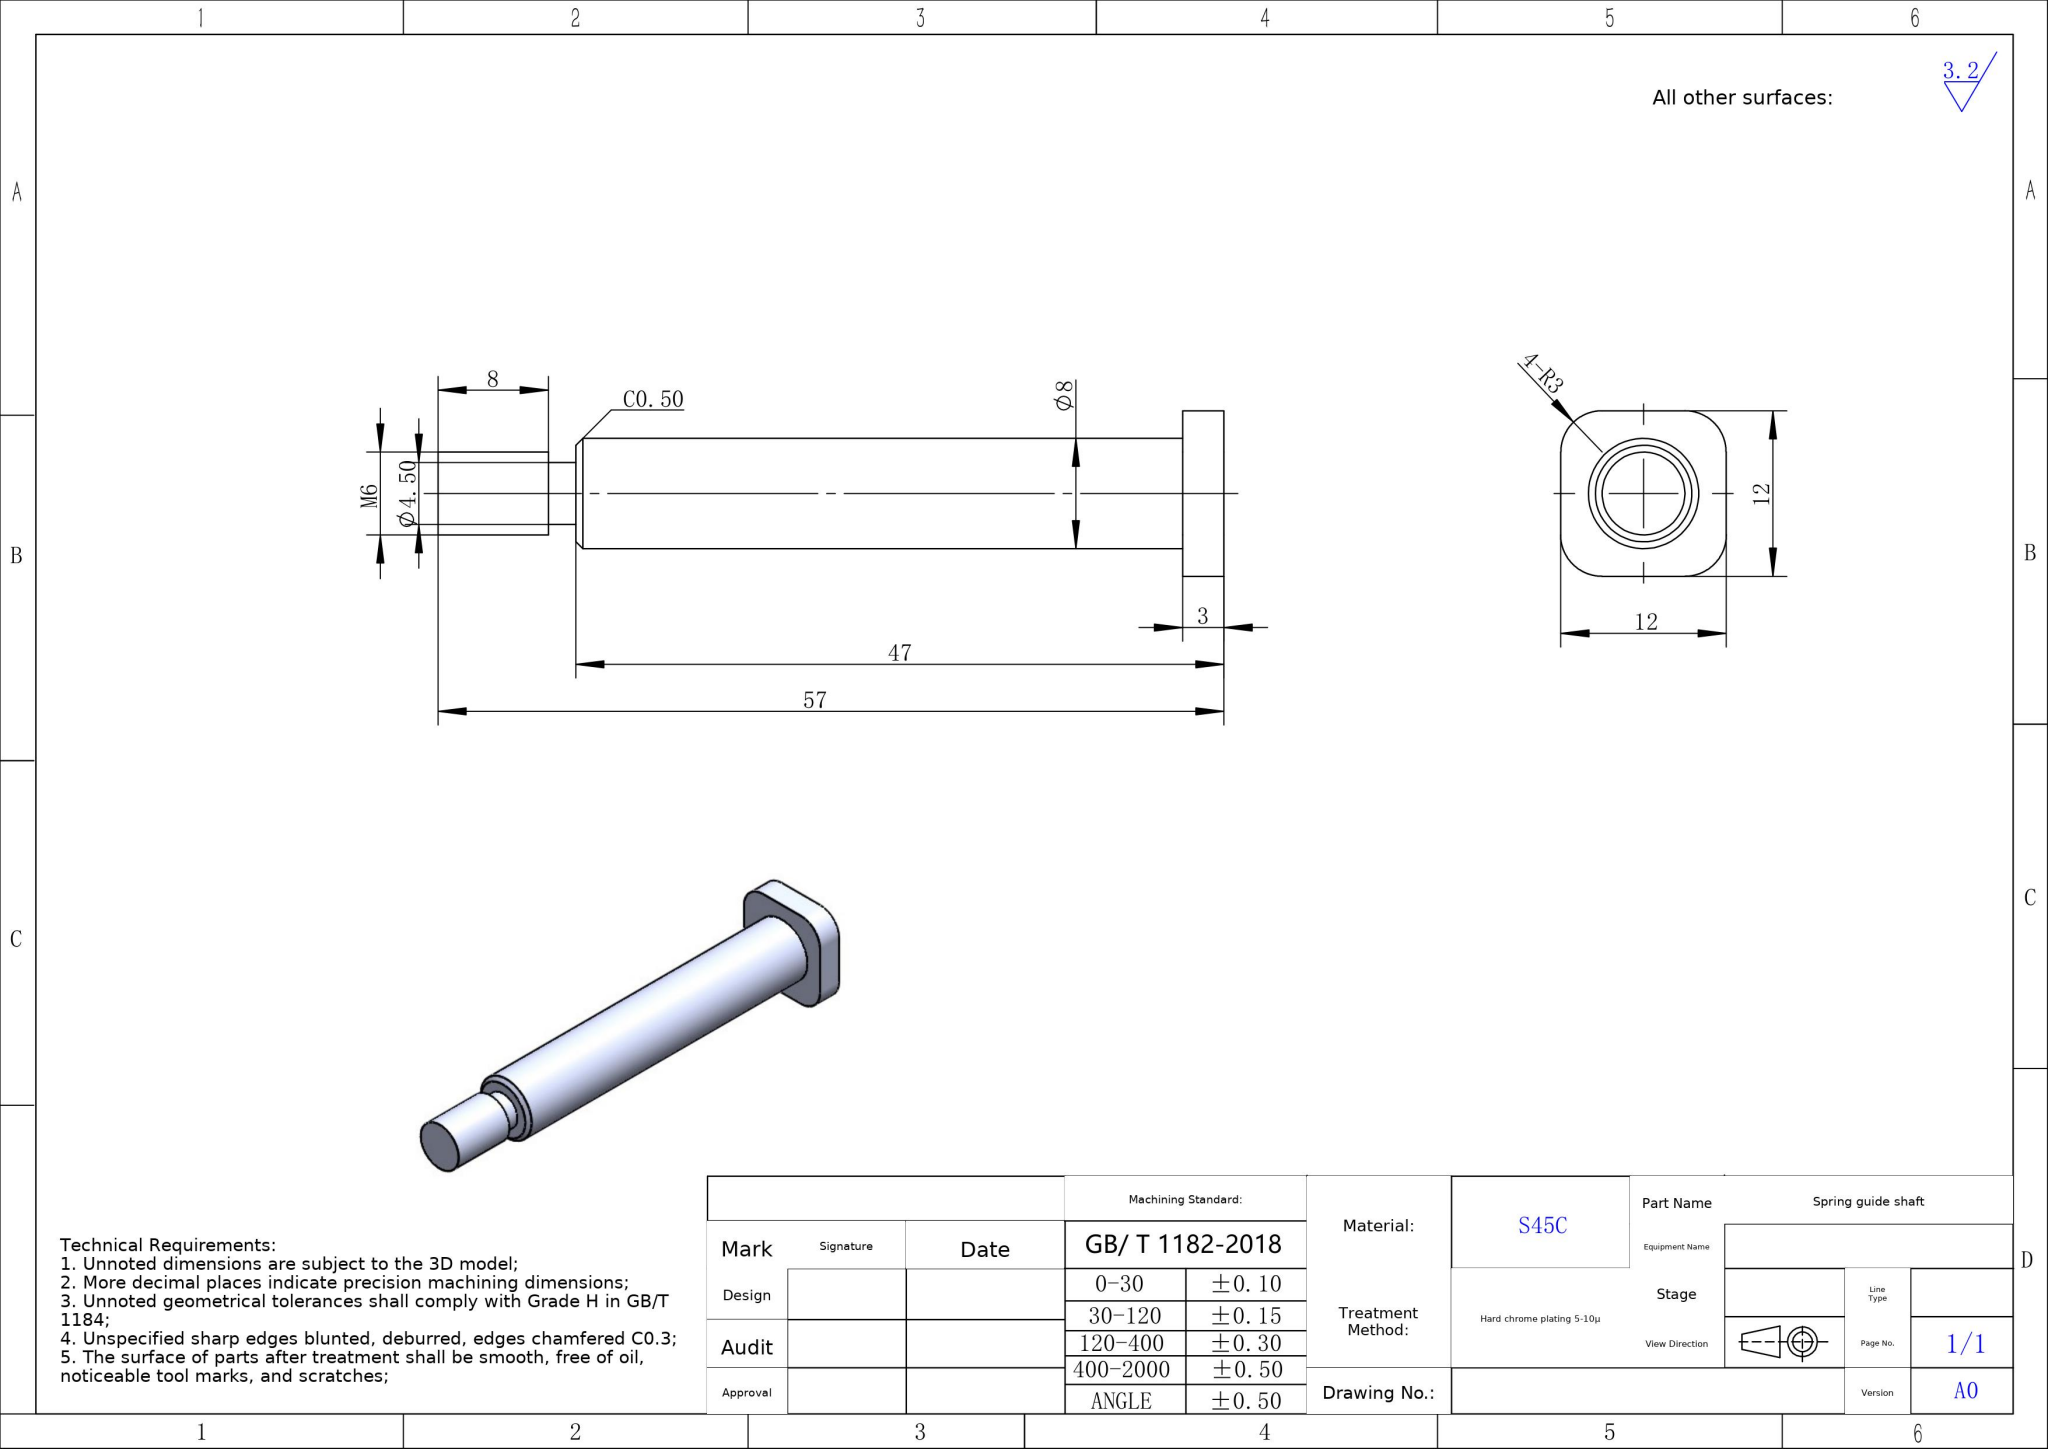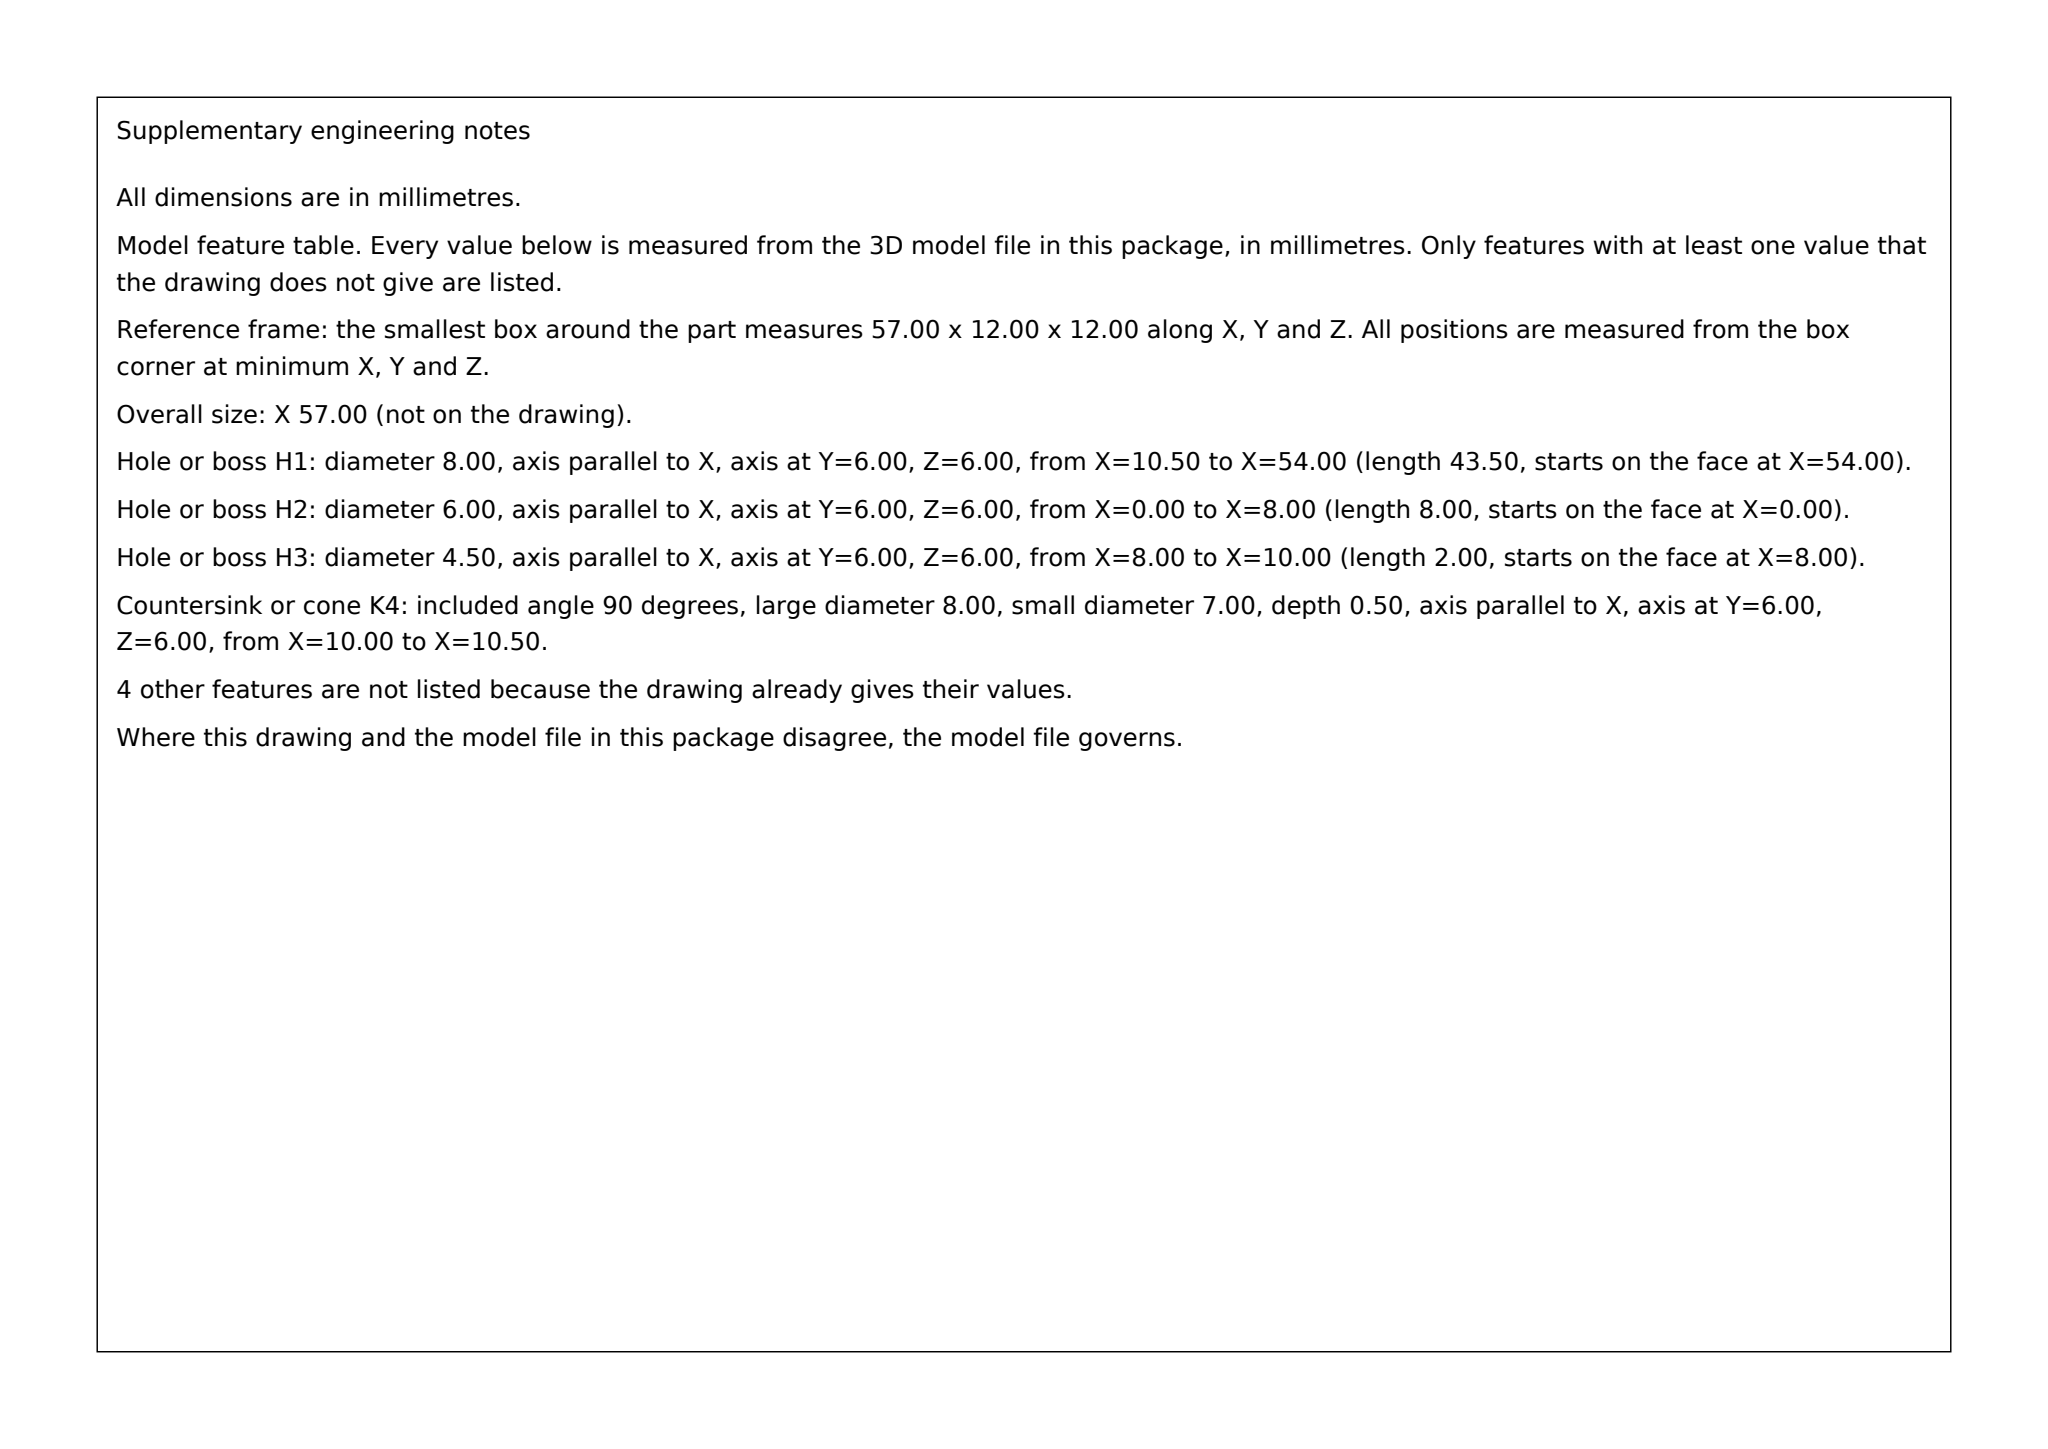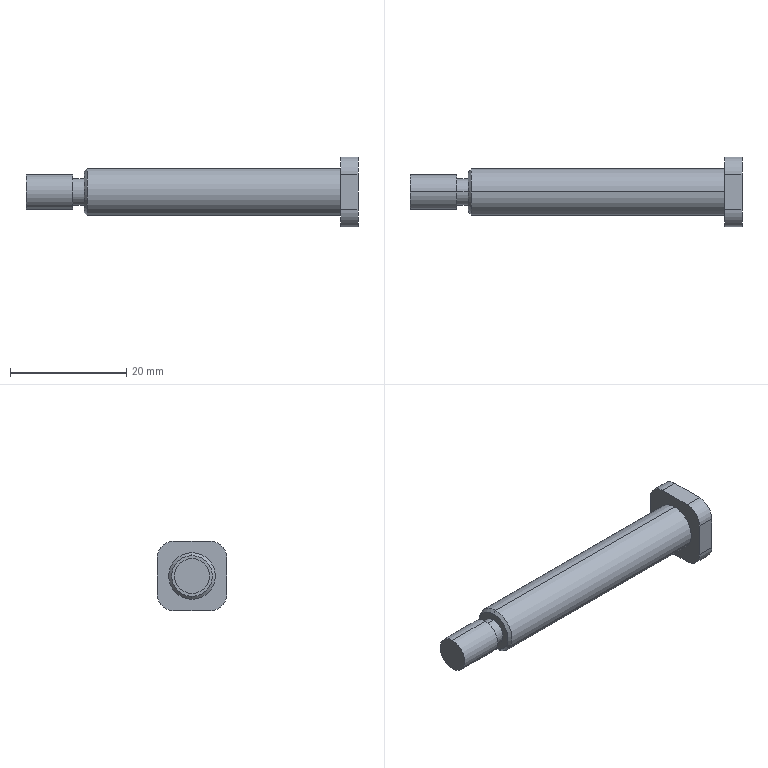Part | SolidWorks | mm | material S45C | 1 solid | 21 faces | box 57 x 12 x 12 mm | volume 2875 mm3 | cylinder 10 | plane 9 | cone 2 | commonest cylinder face diameters 6 x6 4.5 x2 8 x2
build123d program:
from build123d import *

# Parameters (mm, degrees)
SKETCH2_W           = 12
SKETCH2_H           = 12
BOSS_EXTRUDE1_DEPTH = 3
FILLET1_R           = 3
CHAMFER1_SIZE       = 0.5


with BuildPart() as part:
    # Sketch1 → Revolve1 (revolve)
    with BuildSketch(Plane.XY, mode=Mode.PRIVATE) as revolve1_sk:
        Polygon((0, 0), (0, 3), (8, 3), (8, 2.25), (10, 2.25), (10, 4), (57, 4), (57, 0), align=None)
    revolve(revolve1_sk.sketch.rotate(Axis((0, 0, 0), (1, 0, 0)), 90), axis=Axis((0, 0, 0), (1, 0, 0)))

    # Sketch2 → Boss-Extrude1 (add)
    with BuildSketch(Plane(origin=(57, 0, 0), x_dir=(0, 0, -1), z_dir=(1, 0, 0))):
        Rectangle(SKETCH2_W, SKETCH2_H)
    extrude(amount=-BOSS_EXTRUDE1_DEPTH)

    # Fillet1
    fillet1_edges = [part.edges().sort_by_distance(p)[0] for p in [
        (55.5, -6, 6),
        (55.5, 6, 6),
        (55.5, 6, -6),
        (55.5, -6, -6),
    ]]
    fillet(fillet1_edges, radius=FILLET1_R)

    # Chamfer1
    chamfer1_edges = [part.edges().sort_by_distance(p)[0] for p in [
        (10, 0, -4),
    ]]
    chamfer(chamfer1_edges, length=CHAMFER1_SIZE)


solid = part.part
STEP:
#1=CARTESIAN_POINT('',(10.,0.,3.5));
#2=VERTEX_POINT('',#1);
#3=CARTESIAN_POINT('',(10.,0.,-3.5));
#4=VERTEX_POINT('',#3);
#5=CARTESIAN_POINT('',(10.,0.,0.));
#6=DIRECTION('',(-1.,0.,0.));
#7=DIRECTION('',(0.,0.,-1.));
#8=AXIS2_PLACEMENT_3D('',#5,#6,#7);
#9=CIRCLE('',#8,3.5);
#10=EDGE_CURVE('',#2,#4,#9,.T.);
#11=ORIENTED_EDGE('',*,*,#10,.F.);
#12=CARTESIAN_POINT('',(10.5,0.,4.));
#13=VERTEX_POINT('',#12);
#14=CARTESIAN_POINT('',(10.,0.,3.5));
#15=DIRECTION('',(0.7071,0.,0.7071));
#16=VECTOR('',#15,1000.);
#17=LINE('',#14,#16);
#18=EDGE_CURVE('',#2,#13,#17,.T.);
#19=ORIENTED_EDGE('',*,*,#18,.T.);
#20=CARTESIAN_POINT('',(10.5,0.,-4.));
#21=VERTEX_POINT('',#20);
#22=CARTESIAN_POINT('',(10.5,0.,0.));
#23=DIRECTION('',(1.,0.,0.));
#24=DIRECTION('',(0.,0.,-1.));
#25=AXIS2_PLACEMENT_3D('',#22,#23,#24);
#26=CIRCLE('',#25,4.);
#27=EDGE_CURVE('',#21,#13,#26,.T.);
#28=ORIENTED_EDGE('',*,*,#27,.F.);
#29=CARTESIAN_POINT('',(10.,0.,-3.5));
#30=DIRECTION('',(0.7071,0.,-0.7071));
#31=VECTOR('',#30,1000.);
#32=LINE('',#29,#31);
#33=EDGE_CURVE('',#4,#21,#32,.T.);
#34=ORIENTED_EDGE('',*,*,#33,.F.);
#35=EDGE_LOOP('',(#11,#19,#28,#34));
#36=FACE_OUTER_BOUND('',#35,.T.);
#37=CARTESIAN_POINT('',(10.,0.,0.));
#38=DIRECTION('',(1.,0.,0.));
#39=DIRECTION('',(0.,0.,-1.));
#40=AXIS2_PLACEMENT_3D('',#37,#38,#39);
#41=CONICAL_SURFACE('',#40,3.5,0.7854);
#42=ADVANCED_FACE('',(#36),#41,.T.);
#43=CARTESIAN_POINT('',(10.,0.,2.25));
#44=VERTEX_POINT('',#43);
#45=CARTESIAN_POINT('',(10.,0.,-2.25));
#46=VERTEX_POINT('',#45);
#47=CARTESIAN_POINT('',(10.,0.,0.));
#48=DIRECTION('',(-1.,0.,0.));
#49=DIRECTION('',(0.,0.,1.));
#50=AXIS2_PLACEMENT_3D('',#47,#48,#49);
#51=CIRCLE('',#50,2.25);
#52=EDGE_CURVE('',#44,#46,#51,.T.);
#53=ORIENTED_EDGE('',*,*,#52,.T.);
#54=CARTESIAN_POINT('',(8.,0.,-2.25));
#55=VERTEX_POINT('',#54);
#56=CARTESIAN_POINT('',(0.,0.,-2.25));
#57=DIRECTION('',(-1.,0.,0.));
#58=VECTOR('',#57,1000.);
#59=LINE('',#56,#58);
#60=EDGE_CURVE('',#46,#55,#59,.T.);
#61=ORIENTED_EDGE('',*,*,#60,.T.);
#62=CARTESIAN_POINT('',(8.,0.,2.25));
#63=VERTEX_POINT('',#62);
#64=CARTESIAN_POINT('',(8.,0.,0.));
#65=DIRECTION('',(-1.,0.,0.));
#66=DIRECTION('',(0.,0.,1.));
#67=AXIS2_PLACEMENT_3D('',#64,#65,#66);
#68=CIRCLE('',#67,2.25);
#69=EDGE_CURVE('',#63,#55,#68,.T.);
#70=ORIENTED_EDGE('',*,*,#69,.F.);
#71=CARTESIAN_POINT('',(0.,0.,2.25));
#72=DIRECTION('',(-1.,0.,0.));
#73=VECTOR('',#72,1000.);
#74=LINE('',#71,#73);
#75=EDGE_CURVE('',#44,#63,#74,.T.);
#76=ORIENTED_EDGE('',*,*,#75,.F.);
#77=EDGE_LOOP('',(#53,#61,#70,#76));
#78=FACE_OUTER_BOUND('',#77,.T.);
#79=CARTESIAN_POINT('',(0.,0.,0.));
#80=DIRECTION('',(-1.,0.,0.));
#81=DIRECTION('',(0.,0.,1.));
#82=AXIS2_PLACEMENT_3D('',#79,#80,#81);
#83=CYLINDRICAL_SURFACE('',#82,2.25);
#84=ADVANCED_FACE('',(#78),#83,.T.);
#85=CARTESIAN_POINT('',(8.,0.,3.));
#86=VERTEX_POINT('',#85);
#87=CARTESIAN_POINT('',(8.,0.,-3.));
#88=VERTEX_POINT('',#87);
#89=CARTESIAN_POINT('',(8.,0.,0.));
#90=DIRECTION('',(-1.,0.,0.));
#91=DIRECTION('',(0.,0.,1.));
#92=AXIS2_PLACEMENT_3D('',#89,#90,#91);
#93=CIRCLE('',#92,3.);
#94=EDGE_CURVE('',#86,#88,#93,.T.);
#95=ORIENTED_EDGE('',*,*,#94,.T.);
#96=CARTESIAN_POINT('',(0.,0.,-3.));
#97=VERTEX_POINT('',#96);
#98=CARTESIAN_POINT('',(0.,0.,-3.));
#99=DIRECTION('',(-1.,0.,0.));
#100=VECTOR('',#99,1000.);
#101=LINE('',#98,#100);
#102=EDGE_CURVE('',#88,#97,#101,.T.);
#103=ORIENTED_EDGE('',*,*,#102,.T.);
#104=CARTESIAN_POINT('',(0.,0.,3.));
#105=VERTEX_POINT('',#104);
#106=CARTESIAN_POINT('',(0.,0.,0.));
#107=DIRECTION('',(-1.,0.,0.));
#108=DIRECTION('',(0.,0.,1.));
#109=AXIS2_PLACEMENT_3D('',#106,#107,#108);
#110=CIRCLE('',#109,3.);
#111=EDGE_CURVE('',#105,#97,#110,.T.);
#112=ORIENTED_EDGE('',*,*,#111,.F.);
#113=CARTESIAN_POINT('',(0.,0.,3.));
#114=DIRECTION('',(-1.,0.,0.));
#115=VECTOR('',#114,1000.);
#116=LINE('',#113,#115);
#117=EDGE_CURVE('',#86,#105,#116,.T.);
#118=ORIENTED_EDGE('',*,*,#117,.F.);
#119=EDGE_LOOP('',(#95,#103,#112,#118));
#120=FACE_OUTER_BOUND('',#119,.T.);
#121=CARTESIAN_POINT('',(0.,0.,0.));
#122=DIRECTION('',(-1.,0.,0.));
#123=DIRECTION('',(0.,0.,1.));
#124=AXIS2_PLACEMENT_3D('',#121,#122,#123);
#125=CYLINDRICAL_SURFACE('',#124,3.);
#126=ADVANCED_FACE('',(#120),#125,.T.);
#127=CARTESIAN_POINT('',(54.,0.,-4.));
#128=VERTEX_POINT('',#127);
#129=CARTESIAN_POINT('',(54.,0.,4.));
#130=VERTEX_POINT('',#129);
#131=CARTESIAN_POINT('',(54.,0.,0.));
#132=DIRECTION('',(1.,0.,0.));
#133=DIRECTION('',(0.,0.,-1.));
#134=AXIS2_PLACEMENT_3D('',#131,#132,#133);
#135=CIRCLE('',#134,4.);
#136=EDGE_CURVE('',#128,#130,#135,.T.);
#137=ORIENTED_EDGE('',*,*,#136,.F.);
#138=CARTESIAN_POINT('',(0.,0.,-4.));
#139=DIRECTION('',(-1.,0.,0.));
#140=VECTOR('',#139,1000.);
#141=LINE('',#138,#140);
#142=EDGE_CURVE('',#128,#21,#141,.T.);
#143=ORIENTED_EDGE('',*,*,#142,.T.);
#144=ORIENTED_EDGE('',*,*,#27,.T.);
#145=CARTESIAN_POINT('',(0.,0.,4.));
#146=DIRECTION('',(-1.,0.,0.));
#147=VECTOR('',#146,1000.);
#148=LINE('',#145,#147);
#149=EDGE_CURVE('',#130,#13,#148,.T.);
#150=ORIENTED_EDGE('',*,*,#149,.F.);
#151=EDGE_LOOP('',(#137,#143,#144,#150));
#152=FACE_OUTER_BOUND('',#151,.T.);
#153=CARTESIAN_POINT('',(0.,0.,0.));
#154=DIRECTION('',(-1.,0.,0.));
#155=DIRECTION('',(0.,0.,1.));
#156=AXIS2_PLACEMENT_3D('',#153,#154,#155);
#157=CYLINDRICAL_SURFACE('',#156,4.);
#158=ADVANCED_FACE('',(#152),#157,.T.);
#159=ORIENTED_EDGE('',*,*,#142,.F.);
#160=CARTESIAN_POINT('',(54.,0.,0.));
#161=DIRECTION('',(1.,0.,0.));
#162=DIRECTION('',(0.,0.,-1.));
#163=AXIS2_PLACEMENT_3D('',#160,#161,#162);
#164=CIRCLE('',#163,4.);
#165=EDGE_CURVE('',#130,#128,#164,.T.);
#166=ORIENTED_EDGE('',*,*,#165,.F.);
#167=ORIENTED_EDGE('',*,*,#149,.T.);
#168=CARTESIAN_POINT('',(10.5,0.,0.));
#169=DIRECTION('',(1.,0.,0.));
#170=DIRECTION('',(0.,0.,-1.));
#171=AXIS2_PLACEMENT_3D('',#168,#169,#170);
#172=CIRCLE('',#171,4.);
#173=EDGE_CURVE('',#13,#21,#172,.T.);
#174=ORIENTED_EDGE('',*,*,#173,.T.);
#175=EDGE_LOOP('',(#159,#166,#167,#174));
#176=FACE_OUTER_BOUND('',#175,.T.);
#177=CARTESIAN_POINT('',(0.,0.,0.));
#178=DIRECTION('',(-1.,0.,0.));
#179=DIRECTION('',(0.,0.,1.));
#180=AXIS2_PLACEMENT_3D('',#177,#178,#179);
#181=CYLINDRICAL_SURFACE('',#180,4.);
#182=ADVANCED_FACE('',(#176),#181,.T.);
#183=ORIENTED_EDGE('',*,*,#111,.T.);
#184=CARTESIAN_POINT('',(0.,0.,0.));
#185=DIRECTION('',(-1.,0.,0.));
#186=DIRECTION('',(0.,0.,1.));
#187=AXIS2_PLACEMENT_3D('',#184,#185,#186);
#188=CIRCLE('',#187,3.);
#189=EDGE_CURVE('',#97,#105,#188,.T.);
#190=ORIENTED_EDGE('',*,*,#189,.T.);
#191=EDGE_LOOP('',(#183,#190));
#192=FACE_OUTER_BOUND('',#191,.T.);
#193=CARTESIAN_POINT('',(0.,0.,0.));
#194=DIRECTION('',(1.,0.,0.));
#195=DIRECTION('',(0.,0.,-1.));
#196=AXIS2_PLACEMENT_3D('',#193,#194,#195);
#197=PLANE('',#196);
#198=ADVANCED_FACE('',(#192),#197,.F.);
#199=ORIENTED_EDGE('',*,*,#102,.F.);
#200=CARTESIAN_POINT('',(8.,0.,0.));
#201=DIRECTION('',(-1.,0.,0.));
#202=DIRECTION('',(0.,0.,1.));
#203=AXIS2_PLACEMENT_3D('',#200,#201,#202);
#204=CIRCLE('',#203,3.);
#205=EDGE_CURVE('',#88,#86,#204,.T.);
#206=ORIENTED_EDGE('',*,*,#205,.T.);
#207=ORIENTED_EDGE('',*,*,#117,.T.);
#208=ORIENTED_EDGE('',*,*,#189,.F.);
#209=EDGE_LOOP('',(#199,#206,#207,#208));
#210=FACE_OUTER_BOUND('',#209,.T.);
#211=CARTESIAN_POINT('',(0.,0.,0.));
#212=DIRECTION('',(-1.,0.,0.));
#213=DIRECTION('',(0.,0.,1.));
#214=AXIS2_PLACEMENT_3D('',#211,#212,#213);
#215=CYLINDRICAL_SURFACE('',#214,3.);
#216=ADVANCED_FACE('',(#210),#215,.T.);
#217=ORIENTED_EDGE('',*,*,#94,.F.);
#218=ORIENTED_EDGE('',*,*,#205,.F.);
#219=EDGE_LOOP('',(#217,#218));
#220=FACE_OUTER_BOUND('',#219,.T.);
#221=ORIENTED_EDGE('',*,*,#69,.T.);
#222=CARTESIAN_POINT('',(8.,0.,0.));
#223=DIRECTION('',(-1.,0.,0.));
#224=DIRECTION('',(0.,0.,1.));
#225=AXIS2_PLACEMENT_3D('',#222,#223,#224);
#226=CIRCLE('',#225,2.25);
#227=EDGE_CURVE('',#55,#63,#226,.T.);
#228=ORIENTED_EDGE('',*,*,#227,.T.);
#229=EDGE_LOOP('',(#221,#228));
#230=FACE_BOUND('',#229,.T.);
#231=CARTESIAN_POINT('',(8.,3.,0.));
#232=DIRECTION('',(-1.,0.,0.));
#233=DIRECTION('',(0.,0.,1.));
#234=AXIS2_PLACEMENT_3D('',#231,#232,#233);
#235=PLANE('',#234);
#236=ADVANCED_FACE('',(#220,#230),#235,.F.);
#237=ORIENTED_EDGE('',*,*,#60,.F.);
#238=CARTESIAN_POINT('',(10.,0.,0.));
#239=DIRECTION('',(-1.,0.,0.));
#240=DIRECTION('',(0.,0.,1.));
#241=AXIS2_PLACEMENT_3D('',#238,#239,#240);
#242=CIRCLE('',#241,2.25);
#243=EDGE_CURVE('',#46,#44,#242,.T.);
#244=ORIENTED_EDGE('',*,*,#243,.T.);
#245=ORIENTED_EDGE('',*,*,#75,.T.);
#246=ORIENTED_EDGE('',*,*,#227,.F.);
#247=EDGE_LOOP('',(#237,#244,#245,#246));
#248=FACE_OUTER_BOUND('',#247,.T.);
#249=CARTESIAN_POINT('',(0.,0.,0.));
#250=DIRECTION('',(-1.,0.,0.));
#251=DIRECTION('',(0.,0.,1.));
#252=AXIS2_PLACEMENT_3D('',#249,#250,#251);
#253=CYLINDRICAL_SURFACE('',#252,2.25);
#254=ADVANCED_FACE('',(#248),#253,.T.);
#255=CARTESIAN_POINT('',(10.,0.,0.));
#256=DIRECTION('',(-1.,0.,0.));
#257=DIRECTION('',(0.,0.,-1.));
#258=AXIS2_PLACEMENT_3D('',#255,#256,#257);
#259=CIRCLE('',#258,3.5);
#260=EDGE_CURVE('',#4,#2,#259,.T.);
#261=ORIENTED_EDGE('',*,*,#260,.T.);
#262=ORIENTED_EDGE('',*,*,#10,.T.);
#263=EDGE_LOOP('',(#261,#262));
#264=FACE_OUTER_BOUND('',#263,.T.);
#265=ORIENTED_EDGE('',*,*,#52,.F.);
#266=ORIENTED_EDGE('',*,*,#243,.F.);
#267=EDGE_LOOP('',(#265,#266));
#268=FACE_BOUND('',#267,.T.);
#269=CARTESIAN_POINT('',(10.,2.25,0.));
#270=DIRECTION('',(1.,0.,0.));
#271=DIRECTION('',(0.,0.,-1.));
#272=AXIS2_PLACEMENT_3D('',#269,#270,#271);
#273=PLANE('',#272);
#274=ADVANCED_FACE('',(#264,#268),#273,.F.);
#275=CARTESIAN_POINT('',(54.,3.,6.));
#276=VERTEX_POINT('',#275);
#277=CARTESIAN_POINT('',(54.,-3.,6.));
#278=VERTEX_POINT('',#277);
#279=CARTESIAN_POINT('',(54.,-6.,6.));
#280=DIRECTION('',(0.,-1.,0.));
#281=VECTOR('',#280,1000.);
#282=LINE('',#279,#281);
#283=EDGE_CURVE('',#276,#278,#282,.T.);
#284=ORIENTED_EDGE('',*,*,#283,.T.);
#285=CARTESIAN_POINT('',(57.,-3.,6.));
#286=VERTEX_POINT('',#285);
#287=CARTESIAN_POINT('',(54.,-3.,6.));
#288=DIRECTION('',(1.,0.,0.));
#289=VECTOR('',#288,1000.);
#290=LINE('',#287,#289);
#291=EDGE_CURVE('',#278,#286,#290,.T.);
#292=ORIENTED_EDGE('',*,*,#291,.T.);
#293=CARTESIAN_POINT('',(57.,3.,6.));
#294=VERTEX_POINT('',#293);
#295=CARTESIAN_POINT('',(57.,-6.,6.));
#296=DIRECTION('',(0.,-1.,0.));
#297=VECTOR('',#296,1000.);
#298=LINE('',#295,#297);
#299=EDGE_CURVE('',#294,#286,#298,.T.);
#300=ORIENTED_EDGE('',*,*,#299,.F.);
#301=CARTESIAN_POINT('',(54.,3.,6.));
#302=DIRECTION('',(-1.,0.,0.));
#303=VECTOR('',#302,1000.);
#304=LINE('',#301,#303);
#305=EDGE_CURVE('',#294,#276,#304,.T.);
#306=ORIENTED_EDGE('',*,*,#305,.T.);
#307=EDGE_LOOP('',(#284,#292,#300,#306));
#308=FACE_OUTER_BOUND('',#307,.T.);
#309=CARTESIAN_POINT('',(54.,-6.,6.));
#310=DIRECTION('',(0.,0.,1.));
#311=DIRECTION('',(1.,0.,0.));
#312=AXIS2_PLACEMENT_3D('',#309,#310,#311);
#313=PLANE('',#312);
#314=ADVANCED_FACE('',(#308),#313,.T.);
#315=CARTESIAN_POINT('',(57.,6.,-3.));
#316=VERTEX_POINT('',#315);
#317=CARTESIAN_POINT('',(57.,6.,3.));
#318=VERTEX_POINT('',#317);
#319=CARTESIAN_POINT('',(57.,6.,-6.));
#320=DIRECTION('',(0.,-0.,1.));
#321=VECTOR('',#320,1000.);
#322=LINE('',#319,#321);
#323=EDGE_CURVE('',#316,#318,#322,.T.);
#324=ORIENTED_EDGE('',*,*,#323,.F.);
#325=CARTESIAN_POINT('',(54.,6.,-3.));
#326=VERTEX_POINT('',#325);
#327=CARTESIAN_POINT('',(54.,6.,-3.));
#328=DIRECTION('',(-1.,0.,0.));
#329=VECTOR('',#328,1000.);
#330=LINE('',#327,#329);
#331=EDGE_CURVE('',#316,#326,#330,.T.);
#332=ORIENTED_EDGE('',*,*,#331,.T.);
#333=CARTESIAN_POINT('',(54.,6.,3.));
#334=VERTEX_POINT('',#333);
#335=CARTESIAN_POINT('',(54.,6.,-6.));
#336=DIRECTION('',(0.,-0.,1.));
#337=VECTOR('',#336,1000.);
#338=LINE('',#335,#337);
#339=EDGE_CURVE('',#326,#334,#338,.T.);
#340=ORIENTED_EDGE('',*,*,#339,.T.);
#341=CARTESIAN_POINT('',(54.,6.,3.));
#342=DIRECTION('',(1.,0.,0.));
#343=VECTOR('',#342,1000.);
#344=LINE('',#341,#343);
#345=EDGE_CURVE('',#334,#318,#344,.T.);
#346=ORIENTED_EDGE('',*,*,#345,.T.);
#347=EDGE_LOOP('',(#324,#332,#340,#346));
#348=FACE_OUTER_BOUND('',#347,.T.);
#349=CARTESIAN_POINT('',(54.,6.,-6.));
#350=DIRECTION('',(0.,1.,0.));
#351=DIRECTION('',(0.,-0.,1.));
#352=AXIS2_PLACEMENT_3D('',#349,#350,#351);
#353=PLANE('',#352);
#354=ADVANCED_FACE('',(#348),#353,.T.);
#355=CARTESIAN_POINT('',(57.,-3.,-6.));
#356=VERTEX_POINT('',#355);
#357=CARTESIAN_POINT('',(57.,3.,-6.));
#358=VERTEX_POINT('',#357);
#359=CARTESIAN_POINT('',(57.,-6.,-6.));
#360=DIRECTION('',(0.,1.,0.));
#361=VECTOR('',#360,1000.);
#362=LINE('',#359,#361);
#363=EDGE_CURVE('',#356,#358,#362,.T.);
#364=ORIENTED_EDGE('',*,*,#363,.F.);
#365=CARTESIAN_POINT('',(54.,-3.,-6.));
#366=VERTEX_POINT('',#365);
#367=CARTESIAN_POINT('',(54.,-3.,-6.));
#368=DIRECTION('',(-1.,0.,0.));
#369=VECTOR('',#368,1000.);
#370=LINE('',#367,#369);
#371=EDGE_CURVE('',#356,#366,#370,.T.);
#372=ORIENTED_EDGE('',*,*,#371,.T.);
#373=CARTESIAN_POINT('',(54.,3.,-6.));
#374=VERTEX_POINT('',#373);
#375=CARTESIAN_POINT('',(54.,-6.,-6.));
#376=DIRECTION('',(0.,1.,0.));
#377=VECTOR('',#376,1000.);
#378=LINE('',#375,#377);
#379=EDGE_CURVE('',#366,#374,#378,.T.);
#380=ORIENTED_EDGE('',*,*,#379,.T.);
#381=CARTESIAN_POINT('',(54.,3.,-6.));
#382=DIRECTION('',(1.,0.,0.));
#383=VECTOR('',#382,1000.);
#384=LINE('',#381,#383);
#385=EDGE_CURVE('',#374,#358,#384,.T.);
#386=ORIENTED_EDGE('',*,*,#385,.T.);
#387=EDGE_LOOP('',(#364,#372,#380,#386));
#388=FACE_OUTER_BOUND('',#387,.T.);
#389=CARTESIAN_POINT('',(54.,-6.,-6.));
#390=DIRECTION('',(0.,0.,-1.));
#391=DIRECTION('',(-1.,0.,0.));
#392=AXIS2_PLACEMENT_3D('',#389,#390,#391);
#393=PLANE('',#392);
#394=ADVANCED_FACE('',(#388),#393,.T.);
#395=CARTESIAN_POINT('',(54.,-6.,3.));
#396=VERTEX_POINT('',#395);
#397=CARTESIAN_POINT('',(54.,-6.,-3.));
#398=VERTEX_POINT('',#397);
#399=CARTESIAN_POINT('',(54.,-6.,-6.));
#400=DIRECTION('',(0.,0.,-1.));
#401=VECTOR('',#400,1000.);
#402=LINE('',#399,#401);
#403=EDGE_CURVE('',#396,#398,#402,.T.);
#404=ORIENTED_EDGE('',*,*,#403,.T.);
#405=CARTESIAN_POINT('',(57.,-6.,-3.));
#406=VERTEX_POINT('',#405);
#407=CARTESIAN_POINT('',(54.,-6.,-3.));
#408=DIRECTION('',(1.,0.,0.));
#409=VECTOR('',#408,1000.);
#410=LINE('',#407,#409);
#411=EDGE_CURVE('',#398,#406,#410,.T.);
#412=ORIENTED_EDGE('',*,*,#411,.T.);
#413=CARTESIAN_POINT('',(57.,-6.,3.));
#414=VERTEX_POINT('',#413);
#415=CARTESIAN_POINT('',(57.,-6.,-6.));
#416=DIRECTION('',(0.,0.,-1.));
#417=VECTOR('',#416,1000.);
#418=LINE('',#415,#417);
#419=EDGE_CURVE('',#414,#406,#418,.T.);
#420=ORIENTED_EDGE('',*,*,#419,.F.);
#421=CARTESIAN_POINT('',(54.,-6.,3.));
#422=DIRECTION('',(-1.,0.,0.));
#423=VECTOR('',#422,1000.);
#424=LINE('',#421,#423);
#425=EDGE_CURVE('',#414,#396,#424,.T.);
#426=ORIENTED_EDGE('',*,*,#425,.T.);
#427=EDGE_LOOP('',(#404,#412,#420,#426));
#428=FACE_OUTER_BOUND('',#427,.T.);
#429=CARTESIAN_POINT('',(54.,-6.,-6.));
#430=DIRECTION('',(0.,-1.,-0.));
#431=DIRECTION('',(0.,0.,-1.));
#432=AXIS2_PLACEMENT_3D('',#429,#430,#431);
#433=PLANE('',#432);
#434=ADVANCED_FACE('',(#428),#433,.T.);
#435=ORIENTED_EDGE('',*,*,#165,.T.);
#436=ORIENTED_EDGE('',*,*,#136,.T.);
#437=EDGE_LOOP('',(#435,#436));
#438=FACE_BOUND('',#437,.T.);
#439=ORIENTED_EDGE('',*,*,#379,.F.);
#440=CARTESIAN_POINT('',(54.,-3.,-3.));
#441=DIRECTION('',(-1.,0.,0.));
#442=DIRECTION('',(0.,0.,-1.));
#443=AXIS2_PLACEMENT_3D('',#440,#441,#442);
#444=CIRCLE('',#443,3.);
#445=EDGE_CURVE('',#366,#398,#444,.T.);
#446=ORIENTED_EDGE('',*,*,#445,.T.);
#447=ORIENTED_EDGE('',*,*,#403,.F.);
#448=CARTESIAN_POINT('',(54.,-3.,3.));
#449=DIRECTION('',(-1.,0.,0.));
#450=DIRECTION('',(0.,0.,-1.));
#451=AXIS2_PLACEMENT_3D('',#448,#449,#450);
#452=CIRCLE('',#451,3.);
#453=EDGE_CURVE('',#396,#278,#452,.T.);
#454=ORIENTED_EDGE('',*,*,#453,.T.);
#455=ORIENTED_EDGE('',*,*,#283,.F.);
#456=CARTESIAN_POINT('',(54.,3.,3.));
#457=DIRECTION('',(-1.,0.,0.));
#458=DIRECTION('',(0.,0.,-1.));
#459=AXIS2_PLACEMENT_3D('',#456,#457,#458);
#460=CIRCLE('',#459,3.);
#461=EDGE_CURVE('',#276,#334,#460,.T.);
#462=ORIENTED_EDGE('',*,*,#461,.T.);
#463=ORIENTED_EDGE('',*,*,#339,.F.);
#464=CARTESIAN_POINT('',(54.,3.,-3.));
#465=DIRECTION('',(-1.,0.,0.));
#466=DIRECTION('',(0.,0.,-1.));
#467=AXIS2_PLACEMENT_3D('',#464,#465,#466);
#468=CIRCLE('',#467,3.);
#469=EDGE_CURVE('',#326,#374,#468,.T.);
#470=ORIENTED_EDGE('',*,*,#469,.T.);
#471=EDGE_LOOP('',(#439,#446,#447,#454,#455,#462,#463,#470));
#472=FACE_OUTER_BOUND('',#471,.T.);
#473=CARTESIAN_POINT('',(54.,0.,0.));
#474=DIRECTION('',(1.,0.,0.));
#475=DIRECTION('',(0.,0.,-1.));
#476=AXIS2_PLACEMENT_3D('',#473,#474,#475);
#477=PLANE('',#476);
#478=ADVANCED_FACE('',(#438,#472),#477,.F.);
#479=ORIENTED_EDGE('',*,*,#419,.T.);
#480=CARTESIAN_POINT('',(57.,-3.,-3.));
#481=DIRECTION('',(1.,0.,0.));
#482=DIRECTION('',(0.,0.,1.));
#483=AXIS2_PLACEMENT_3D('',#480,#481,#482);
#484=CIRCLE('',#483,3.);
#485=EDGE_CURVE('',#406,#356,#484,.T.);
#486=ORIENTED_EDGE('',*,*,#485,.T.);
#487=ORIENTED_EDGE('',*,*,#363,.T.);
#488=CARTESIAN_POINT('',(57.,3.,-3.));
#489=DIRECTION('',(1.,0.,0.));
#490=DIRECTION('',(0.,0.,1.));
#491=AXIS2_PLACEMENT_3D('',#488,#489,#490);
#492=CIRCLE('',#491,3.);
#493=EDGE_CURVE('',#358,#316,#492,.T.);
#494=ORIENTED_EDGE('',*,*,#493,.T.);
#495=ORIENTED_EDGE('',*,*,#323,.T.);
#496=CARTESIAN_POINT('',(57.,3.,3.));
#497=DIRECTION('',(1.,0.,0.));
#498=DIRECTION('',(0.,-0.,1.));
#499=AXIS2_PLACEMENT_3D('',#496,#497,#498);
#500=CIRCLE('',#499,3.);
#501=EDGE_CURVE('',#318,#294,#500,.T.);
#502=ORIENTED_EDGE('',*,*,#501,.T.);
#503=ORIENTED_EDGE('',*,*,#299,.T.);
#504=CARTESIAN_POINT('',(57.,-3.,3.));
#505=DIRECTION('',(1.,0.,0.));
#506=DIRECTION('',(0.,0.,1.));
#507=AXIS2_PLACEMENT_3D('',#504,#505,#506);
#508=CIRCLE('',#507,3.);
#509=EDGE_CURVE('',#286,#414,#508,.T.);
#510=ORIENTED_EDGE('',*,*,#509,.T.);
#511=EDGE_LOOP('',(#479,#486,#487,#494,#495,#502,#503,#510));
#512=FACE_OUTER_BOUND('',#511,.T.);
#513=CARTESIAN_POINT('',(57.,4.,0.));
#514=DIRECTION('',(-1.,0.,0.));
#515=DIRECTION('',(0.,0.,1.));
#516=AXIS2_PLACEMENT_3D('',#513,#514,#515);
#517=PLANE('',#516);
#518=ADVANCED_FACE('',(#512),#517,.F.);
#519=ORIENTED_EDGE('',*,*,#445,.F.);
#520=ORIENTED_EDGE('',*,*,#371,.F.);
#521=ORIENTED_EDGE('',*,*,#485,.F.);
#522=ORIENTED_EDGE('',*,*,#411,.F.);
#523=EDGE_LOOP('',(#519,#520,#521,#522));
#524=FACE_OUTER_BOUND('',#523,.T.);
#525=CARTESIAN_POINT('',(54.,-3.,-3.));
#526=DIRECTION('',(1.,0.,0.));
#527=DIRECTION('',(0.,0.,-1.));
#528=AXIS2_PLACEMENT_3D('',#525,#526,#527);
#529=CYLINDRICAL_SURFACE('',#528,3.);
#530=ADVANCED_FACE('',(#524),#529,.T.);
#531=ORIENTED_EDGE('',*,*,#453,.F.);
#532=ORIENTED_EDGE('',*,*,#425,.F.);
#533=ORIENTED_EDGE('',*,*,#509,.F.);
#534=ORIENTED_EDGE('',*,*,#291,.F.);
#535=EDGE_LOOP('',(#531,#532,#533,#534));
#536=FACE_OUTER_BOUND('',#535,.T.);
#537=CARTESIAN_POINT('',(54.,-3.,3.));
#538=DIRECTION('',(1.,0.,0.));
#539=DIRECTION('',(0.,0.,-1.));
#540=AXIS2_PLACEMENT_3D('',#537,#538,#539);
#541=CYLINDRICAL_SURFACE('',#540,3.);
#542=ADVANCED_FACE('',(#536),#541,.T.);
#543=ORIENTED_EDGE('',*,*,#469,.F.);
#544=ORIENTED_EDGE('',*,*,#331,.F.);
#545=ORIENTED_EDGE('',*,*,#493,.F.);
#546=ORIENTED_EDGE('',*,*,#385,.F.);
#547=EDGE_LOOP('',(#543,#544,#545,#546));
#548=FACE_OUTER_BOUND('',#547,.T.);
#549=CARTESIAN_POINT('',(54.,3.,-3.));
#550=DIRECTION('',(1.,0.,0.));
#551=DIRECTION('',(0.,0.,-1.));
#552=AXIS2_PLACEMENT_3D('',#549,#550,#551);
#553=CYLINDRICAL_SURFACE('',#552,3.);
#554=ADVANCED_FACE('',(#548),#553,.T.);
#555=ORIENTED_EDGE('',*,*,#461,.F.);
#556=ORIENTED_EDGE('',*,*,#305,.F.);
#557=ORIENTED_EDGE('',*,*,#501,.F.);
#558=ORIENTED_EDGE('',*,*,#345,.F.);
#559=EDGE_LOOP('',(#555,#556,#557,#558));
#560=FACE_OUTER_BOUND('',#559,.T.);
#561=CARTESIAN_POINT('',(54.,3.,3.));
#562=DIRECTION('',(1.,0.,0.));
#563=DIRECTION('',(0.,0.,-1.));
#564=AXIS2_PLACEMENT_3D('',#561,#562,#563);
#565=CYLINDRICAL_SURFACE('',#564,3.);
#566=ADVANCED_FACE('',(#560),#565,.T.);
#567=ORIENTED_EDGE('',*,*,#18,.F.);
#568=ORIENTED_EDGE('',*,*,#260,.F.);
#569=ORIENTED_EDGE('',*,*,#33,.T.);
#570=ORIENTED_EDGE('',*,*,#173,.F.);
#571=EDGE_LOOP('',(#567,#568,#569,#570));
#572=FACE_OUTER_BOUND('',#571,.T.);
#573=CARTESIAN_POINT('',(10.,0.,0.));
#574=DIRECTION('',(1.,0.,0.));
#575=DIRECTION('',(0.,0.,-1.));
#576=AXIS2_PLACEMENT_3D('',#573,#574,#575);
#577=CONICAL_SURFACE('',#576,3.5,0.7854);
#578=ADVANCED_FACE('',(#572),#577,.T.);
#579=CLOSED_SHELL('',(#42,#84,#126,#158,#182,#198,#216,#236,#254,#274,#314,#354,#394,#434,#478,#518,#530,#542,#554,#566,#578));
#580=MANIFOLD_SOLID_BREP('',#579);
#581=CARTESIAN_POINT('',(0.,0.,0.));
#582=DIRECTION('',(0.,0.,1.));
#583=DIRECTION('',(1.,0.,0.));
#584=AXIS2_PLACEMENT_3D('',#581,#582,#583);
#585=(LENGTH_UNIT()NAMED_UNIT(*)SI_UNIT(.MILLI.,.METRE.));
#586=UNCERTAINTY_MEASURE_WITH_UNIT(LENGTH_MEASURE(0.00001),#585,'','');
#587=(NAMED_UNIT(*)PLANE_ANGLE_UNIT()SI_UNIT($,.RADIAN.));
#588=(NAMED_UNIT(*)SI_UNIT($,.STERADIAN.)SOLID_ANGLE_UNIT());
#589=(GEOMETRIC_REPRESENTATION_CONTEXT(3)GLOBAL_UNCERTAINTY_ASSIGNED_CONTEXT((#586))GLOBAL_UNIT_ASSIGNED_CONTEXT((#585,#587,#588))REPRESENTATION_CONTEXT('',''));
#590=ADVANCED_BREP_SHAPE_REPRESENTATION('',(#580,#584),#589);